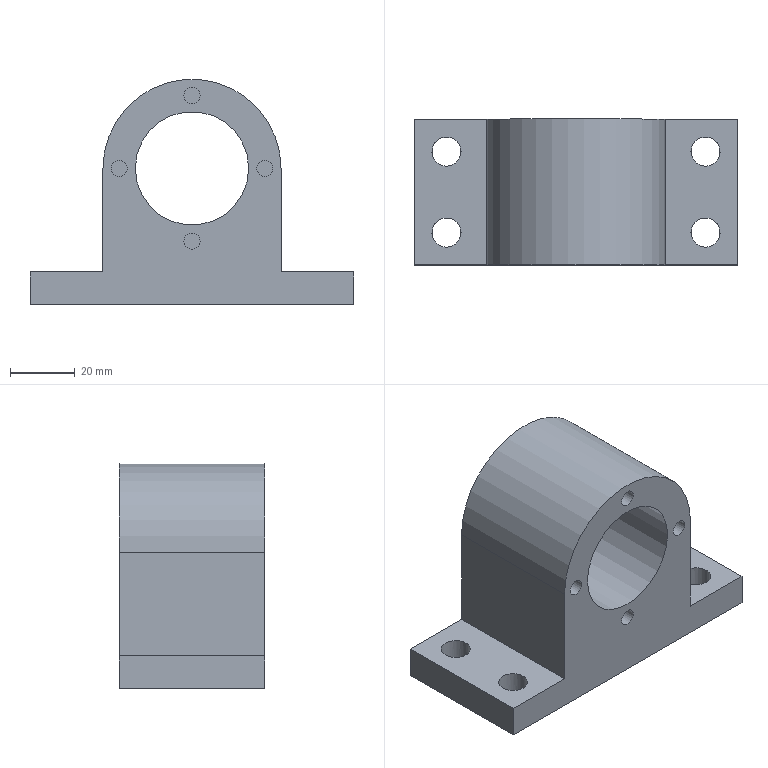Component | NX | BEARING_BLOCK_4 | 1 solid | 31 faces | volume 129146 mm3 | plane 17 | cylinder 14 | commonest cylinder face diameters 5 x8 9 x4 55 x1 35 x1